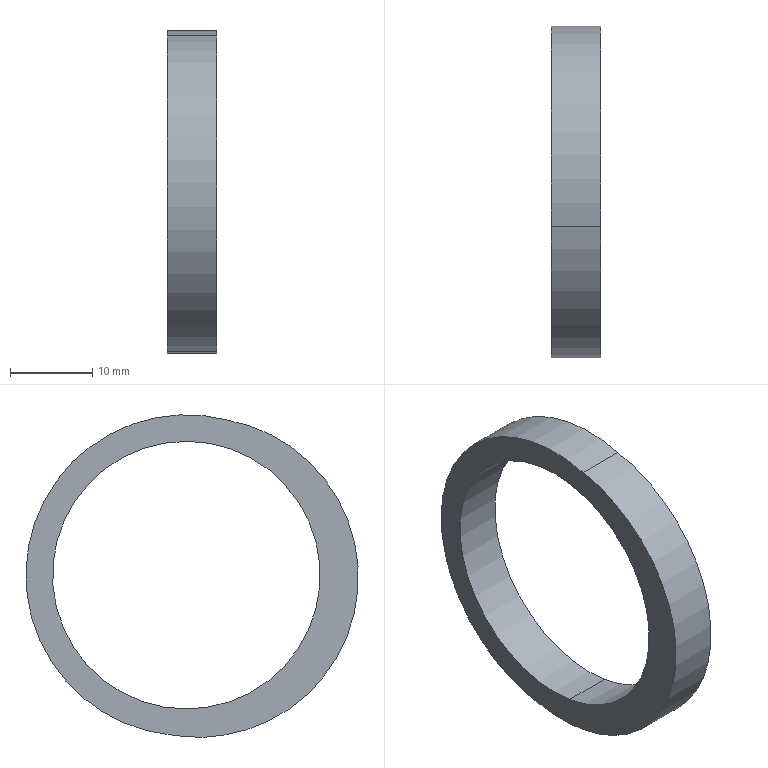Component | SolidWorks | OriginalWasher-1 | 1 solid | 7 faces | box 6 x 40.52 x 39.32 mm | volume 2523 mm3 | cylinder 5 | plane 2 | commonest cylinder face diameters 32.621 x2 39 x2 39.114 x1
build123d program:
from build123d import *

# Parameters (mm, degrees)
SKETCH2_R           = 16.311
BOSS_EXTRUDE1_DEPTH = 3
SKETCH3_R           = 16.311
BOSS_EXTRUDE2_DEPTH = 3


with BuildPart() as part:
    # Sketch2 → Boss-Extrude1 (new body)
    with BuildSketch(Plane.XY.offset(-0.15)):
        with BuildLine():
            ThreePointArc((18.395, 53.747), (6.985, 80.072), (-18.395, 66.691))
            ThreePointArc((-18.395, 66.691), (-6.472, 41.824), (18.395, 53.747))
        make_face()
        with Locations((0.4943, 61.624)):
            Circle(SKETCH2_R, mode=Mode.SUBTRACT)
    extrude(amount=BOSS_EXTRUDE1_DEPTH)

    # Sketch3 → Boss-Extrude2 (add)
    with BuildSketch(Plane.XY.offset(2.85)):
        with BuildLine():
            ThreePointArc((18.395, 53.747), (6.985, 80.072), (-18.395, 66.691))
            ThreePointArc((-18.395, 66.691), (-6.472, 41.824), (18.395, 53.747))
        make_face()
        with Locations((0.4943, 61.624)):
            Circle(SKETCH3_R, mode=Mode.SUBTRACT)
    extrude(amount=BOSS_EXTRUDE2_DEPTH)


solid = part.part

# Placed as in the assembly
solid = solid.moved(Location((-173.15, -0.6926, 9.357), (-9.192, -90, 0)))
STEP:
#1=COLOUR_RGB('',0.7922,0.8196,0.9333);
#2=FILL_AREA_STYLE_COLOUR('',#1);
#3=FILL_AREA_STYLE('',(#2));
#4=SURFACE_STYLE_FILL_AREA(#3);
#5=SURFACE_SIDE_STYLE('',(#4));
#6=SURFACE_STYLE_USAGE(.BOTH.,#5);
#7=PRESENTATION_STYLE_ASSIGNMENT((#6));
#8=CARTESIAN_POINT('',(-7.047,2.268,-0.6339));
#9=VERTEX_POINT('',#8);
#10=CARTESIAN_POINT('',(-7.047,2.473,0.6339));
#11=VERTEX_POINT('',#10);
#12=CARTESIAN_POINT('',(-7.047,2.371,-0.));
#13=DIRECTION('',(-1.,0.,0.));
#14=DIRECTION('',(0.,0.1598,0.9872));
#15=AXIS2_PLACEMENT_3D('',#12,#13,#14);
#16=CIRCLE('',#15,0.6421);
#17=EDGE_CURVE('',#9,#11,#16,.T.);
#18=ORIENTED_EDGE('',*,*,#17,.T.);
#19=CARTESIAN_POINT('',(-6.811,2.473,0.6339));
#20=VERTEX_POINT('',#19);
#21=CARTESIAN_POINT('',(-6.929,2.473,0.6339));
#22=DIRECTION('',(1.,0.,0.));
#23=VECTOR('',#22,39.37);
#24=LINE('',#21,#23);
#25=EDGE_CURVE('',#11,#20,#24,.T.);
#26=ORIENTED_EDGE('',*,*,#25,.T.);
#27=CARTESIAN_POINT('',(-6.811,2.268,-0.6339));
#28=VERTEX_POINT('',#27);
#29=CARTESIAN_POINT('',(-6.811,2.371,-0.));
#30=DIRECTION('',(-1.,0.,0.));
#31=DIRECTION('',(0.,0.1598,0.9872));
#32=AXIS2_PLACEMENT_3D('',#29,#30,#31);
#33=CIRCLE('',#32,0.6421);
#34=EDGE_CURVE('',#28,#20,#33,.T.);
#35=ORIENTED_EDGE('',*,*,#34,.F.);
#36=CARTESIAN_POINT('',(-6.929,2.268,-0.6339));
#37=DIRECTION('',(1.,0.,0.));
#38=VECTOR('',#37,39.37);
#39=LINE('',#36,#38);
#40=EDGE_CURVE('',#9,#28,#39,.T.);
#41=ORIENTED_EDGE('',*,*,#40,.F.);
#42=EDGE_LOOP('',(#18,#26,#35,#41));
#43=FACE_OUTER_BOUND('',#42,.T.);
#44=CARTESIAN_POINT('',(-6.929,2.371,-0.));
#45=DIRECTION('',(1.,0.,0.));
#46=DIRECTION('',(0.,-0.1598,-0.9872));
#47=AXIS2_PLACEMENT_3D('',#44,#45,#46);
#48=CYLINDRICAL_SURFACE('',#47,0.6421);
#49=ADVANCED_FACE('',(#43),#48,.F.);
#50=CARTESIAN_POINT('',(-7.047,2.19,-0.7682));
#51=VERTEX_POINT('',#50);
#52=CARTESIAN_POINT('',(-7.047,2.177,0.7452));
#53=VERTEX_POINT('',#52);
#54=CARTESIAN_POINT('',(-7.047,2.313,-0.01038));
#55=DIRECTION('',(-1.,0.,0.));
#56=DIRECTION('',(0.,0.1598,0.9872));
#57=AXIS2_PLACEMENT_3D('',#54,#55,#56);
#58=CIRCLE('',#57,0.7677);
#59=EDGE_CURVE('',#51,#53,#58,.T.);
#60=ORIENTED_EDGE('',*,*,#59,.F.);
#61=CARTESIAN_POINT('',(-6.811,2.19,-0.7682));
#62=VERTEX_POINT('',#61);
#63=CARTESIAN_POINT('',(-6.929,2.19,-0.7682));
#64=DIRECTION('',(1.,0.,0.));
#65=VECTOR('',#64,39.37);
#66=LINE('',#63,#65);
#67=EDGE_CURVE('',#51,#62,#66,.T.);
#68=ORIENTED_EDGE('',*,*,#67,.T.);
#69=CARTESIAN_POINT('',(-6.811,2.177,0.7452));
#70=VERTEX_POINT('',#69);
#71=CARTESIAN_POINT('',(-6.811,2.313,-0.01038));
#72=DIRECTION('',(-1.,0.,0.));
#73=DIRECTION('',(0.,0.1598,0.9872));
#74=AXIS2_PLACEMENT_3D('',#71,#72,#73);
#75=CIRCLE('',#74,0.7677);
#76=EDGE_CURVE('',#62,#70,#75,.T.);
#77=ORIENTED_EDGE('',*,*,#76,.T.);
#78=CARTESIAN_POINT('',(-6.929,2.177,0.7452));
#79=DIRECTION('',(1.,0.,0.));
#80=VECTOR('',#79,39.37);
#81=LINE('',#78,#80);
#82=EDGE_CURVE('',#53,#70,#81,.T.);
#83=ORIENTED_EDGE('',*,*,#82,.F.);
#84=EDGE_LOOP('',(#60,#68,#77,#83));
#85=FACE_OUTER_BOUND('',#84,.T.);
#86=CARTESIAN_POINT('',(-6.929,2.313,-0.01038));
#87=DIRECTION('',(1.,0.,0.));
#88=DIRECTION('',(0.,-0.1598,-0.9872));
#89=AXIS2_PLACEMENT_3D('',#86,#87,#88);
#90=CYLINDRICAL_SURFACE('',#89,0.7677);
#91=ADVANCED_FACE('',(#85),#90,.T.);
#92=CARTESIAN_POINT('',(-6.811,2.449,-0.766));
#93=VERTEX_POINT('',#92);
#94=CARTESIAN_POINT('',(-6.811,2.313,-0.01038));
#95=DIRECTION('',(-1.,0.,0.));
#96=DIRECTION('',(0.,0.1598,0.9872));
#97=AXIS2_PLACEMENT_3D('',#94,#95,#96);
#98=CIRCLE('',#97,0.7677);
#99=EDGE_CURVE('',#93,#62,#98,.T.);
#100=ORIENTED_EDGE('',*,*,#99,.F.);
#101=CARTESIAN_POINT('',(-6.811,2.371,-0.));
#102=DIRECTION('',(-1.,0.,0.));
#103=DIRECTION('',(0.,0.1598,0.9872));
#104=AXIS2_PLACEMENT_3D('',#101,#102,#103);
#105=CIRCLE('',#104,0.77);
#106=EDGE_CURVE('',#70,#93,#105,.T.);
#107=ORIENTED_EDGE('',*,*,#106,.F.);
#108=ORIENTED_EDGE('',*,*,#76,.F.);
#109=EDGE_LOOP('',(#100,#107,#108));
#110=FACE_OUTER_BOUND('',#109,.T.);
#111=ORIENTED_EDGE('',*,*,#34,.T.);
#112=CARTESIAN_POINT('',(-6.811,2.371,-0.));
#113=DIRECTION('',(-1.,0.,0.));
#114=DIRECTION('',(0.,0.1598,0.9872));
#115=AXIS2_PLACEMENT_3D('',#112,#113,#114);
#116=CIRCLE('',#115,0.6421);
#117=EDGE_CURVE('',#20,#28,#116,.T.);
#118=ORIENTED_EDGE('',*,*,#117,.T.);
#119=EDGE_LOOP('',(#111,#118));
#120=FACE_BOUND('',#119,.T.);
#121=CARTESIAN_POINT('',(-6.811,2.342,-0.005188));
#122=DIRECTION('',(-1.,0.,0.));
#123=DIRECTION('',(0.,0.1598,0.9872));
#124=AXIS2_PLACEMENT_3D('',#121,#122,#123);
#125=PLANE('',#124);
#126=ADVANCED_FACE('',(#110,#120),#125,.F.);
#127=ORIENTED_EDGE('',*,*,#67,.F.);
#128=CARTESIAN_POINT('',(-7.047,2.449,-0.766));
#129=VERTEX_POINT('',#128);
#130=CARTESIAN_POINT('',(-7.047,2.313,-0.01038));
#131=DIRECTION('',(-1.,0.,0.));
#132=DIRECTION('',(0.,0.1598,0.9872));
#133=AXIS2_PLACEMENT_3D('',#130,#131,#132);
#134=CIRCLE('',#133,0.7677);
#135=EDGE_CURVE('',#129,#51,#134,.T.);
#136=ORIENTED_EDGE('',*,*,#135,.F.);
#137=CARTESIAN_POINT('',(-6.929,2.449,-0.766));
#138=DIRECTION('',(1.,0.,0.));
#139=VECTOR('',#138,39.37);
#140=LINE('',#137,#139);
#141=EDGE_CURVE('',#129,#93,#140,.T.);
#142=ORIENTED_EDGE('',*,*,#141,.T.);
#143=ORIENTED_EDGE('',*,*,#99,.T.);
#144=EDGE_LOOP('',(#127,#136,#142,#143));
#145=FACE_OUTER_BOUND('',#144,.T.);
#146=CARTESIAN_POINT('',(-6.929,2.313,-0.01038));
#147=DIRECTION('',(1.,0.,0.));
#148=DIRECTION('',(0.,-0.1598,-0.9872));
#149=AXIS2_PLACEMENT_3D('',#146,#147,#148);
#150=CYLINDRICAL_SURFACE('',#149,0.7677);
#151=ADVANCED_FACE('',(#145),#150,.T.);
#152=ORIENTED_EDGE('',*,*,#106,.T.);
#153=ORIENTED_EDGE('',*,*,#141,.F.);
#154=CARTESIAN_POINT('',(-7.047,2.371,-0.));
#155=DIRECTION('',(-1.,0.,0.));
#156=DIRECTION('',(0.,0.1598,0.9872));
#157=AXIS2_PLACEMENT_3D('',#154,#155,#156);
#158=CIRCLE('',#157,0.77);
#159=EDGE_CURVE('',#53,#129,#158,.T.);
#160=ORIENTED_EDGE('',*,*,#159,.F.);
#161=ORIENTED_EDGE('',*,*,#82,.T.);
#162=EDGE_LOOP('',(#152,#153,#160,#161));
#163=FACE_OUTER_BOUND('',#162,.T.);
#164=CARTESIAN_POINT('',(-6.929,2.371,-0.));
#165=DIRECTION('',(1.,0.,0.));
#166=DIRECTION('',(0.,-0.1598,-0.9872));
#167=AXIS2_PLACEMENT_3D('',#164,#165,#166);
#168=CYLINDRICAL_SURFACE('',#167,0.77);
#169=ADVANCED_FACE('',(#163),#168,.T.);
#170=ORIENTED_EDGE('',*,*,#25,.F.);
#171=CARTESIAN_POINT('',(-7.047,2.371,-0.));
#172=DIRECTION('',(-1.,0.,0.));
#173=DIRECTION('',(0.,0.1598,0.9872));
#174=AXIS2_PLACEMENT_3D('',#171,#172,#173);
#175=CIRCLE('',#174,0.6421);
#176=EDGE_CURVE('',#11,#9,#175,.T.);
#177=ORIENTED_EDGE('',*,*,#176,.T.);
#178=ORIENTED_EDGE('',*,*,#40,.T.);
#179=ORIENTED_EDGE('',*,*,#117,.F.);
#180=EDGE_LOOP('',(#170,#177,#178,#179));
#181=FACE_OUTER_BOUND('',#180,.T.);
#182=CARTESIAN_POINT('',(-6.929,2.371,-0.));
#183=DIRECTION('',(1.,0.,0.));
#184=DIRECTION('',(0.,-0.1598,-0.9872));
#185=AXIS2_PLACEMENT_3D('',#182,#183,#184);
#186=CYLINDRICAL_SURFACE('',#185,0.6421);
#187=ADVANCED_FACE('',(#181),#186,.F.);
#188=ORIENTED_EDGE('',*,*,#135,.T.);
#189=ORIENTED_EDGE('',*,*,#59,.T.);
#190=ORIENTED_EDGE('',*,*,#159,.T.);
#191=EDGE_LOOP('',(#188,#189,#190));
#192=FACE_OUTER_BOUND('',#191,.T.);
#193=ORIENTED_EDGE('',*,*,#17,.F.);
#194=ORIENTED_EDGE('',*,*,#176,.F.);
#195=EDGE_LOOP('',(#193,#194));
#196=FACE_BOUND('',#195,.T.);
#197=CARTESIAN_POINT('',(-7.047,2.342,-0.005188));
#198=DIRECTION('',(-1.,0.,0.));
#199=DIRECTION('',(0.,0.1598,0.9872));
#200=AXIS2_PLACEMENT_3D('',#197,#198,#199);
#201=PLANE('',#200);
#202=ADVANCED_FACE('',(#192,#196),#201,.T.);
#203=CLOSED_SHELL('',(#49,#91,#126,#151,#169,#187,#202));
#204=MANIFOLD_SOLID_BREP('',#203);
#205=STYLED_ITEM('',(#7),#204);
#206=(LENGTH_UNIT()NAMED_UNIT(*)SI_UNIT($,.METRE.));
#207=LENGTH_MEASURE_WITH_UNIT(LENGTH_MEASURE(0.0254),#206);
#208=DIMENSIONAL_EXPONENTS(1.,0.,0.,0.,0.,0.,0.);
#209=(CONVERSION_BASED_UNIT('',#207)LENGTH_UNIT()NAMED_UNIT(#208));
#210=UNCERTAINTY_MEASURE_WITH_UNIT(LENGTH_MEASURE(0.00001),#209,'','');
#211=(NAMED_UNIT(*)PLANE_ANGLE_UNIT()SI_UNIT($,.RADIAN.));
#212=(NAMED_UNIT(*)SI_UNIT($,.STERADIAN.)SOLID_ANGLE_UNIT());
#213=(GEOMETRIC_REPRESENTATION_CONTEXT(3)GLOBAL_UNCERTAINTY_ASSIGNED_CONTEXT((#210))GLOBAL_UNIT_ASSIGNED_CONTEXT((#209,#211,#212))REPRESENTATION_CONTEXT('',''));
#214=MECHANICAL_DESIGN_GEOMETRIC_PRESENTATION_REPRESENTATION('',(#205),#213);
#215=CARTESIAN_POINT('',(0.,0.,0.));
#216=DIRECTION('',(0.,0.,1.));
#217=DIRECTION('',(1.,0.,0.));
#218=AXIS2_PLACEMENT_3D('',#215,#216,#217);
#219=(LENGTH_UNIT()NAMED_UNIT(*)SI_UNIT($,.METRE.));
#220=LENGTH_MEASURE_WITH_UNIT(LENGTH_MEASURE(0.0254),#219);
#221=DIMENSIONAL_EXPONENTS(1.,0.,0.,0.,0.,0.,0.);
#222=(CONVERSION_BASED_UNIT('',#220)LENGTH_UNIT()NAMED_UNIT(#221));
#223=UNCERTAINTY_MEASURE_WITH_UNIT(LENGTH_MEASURE(0.00001),#222,'','');
#224=(NAMED_UNIT(*)PLANE_ANGLE_UNIT()SI_UNIT($,.RADIAN.));
#225=(NAMED_UNIT(*)SI_UNIT($,.STERADIAN.)SOLID_ANGLE_UNIT());
#226=(GEOMETRIC_REPRESENTATION_CONTEXT(3)GLOBAL_UNCERTAINTY_ASSIGNED_CONTEXT((#223))GLOBAL_UNIT_ASSIGNED_CONTEXT((#222,#224,#225))REPRESENTATION_CONTEXT('',''));
#227=ADVANCED_BREP_SHAPE_REPRESENTATION('',(#204,#218),#226);
#228=PRESENTATION_LAYER_ASSIGNMENT('','',(#205));